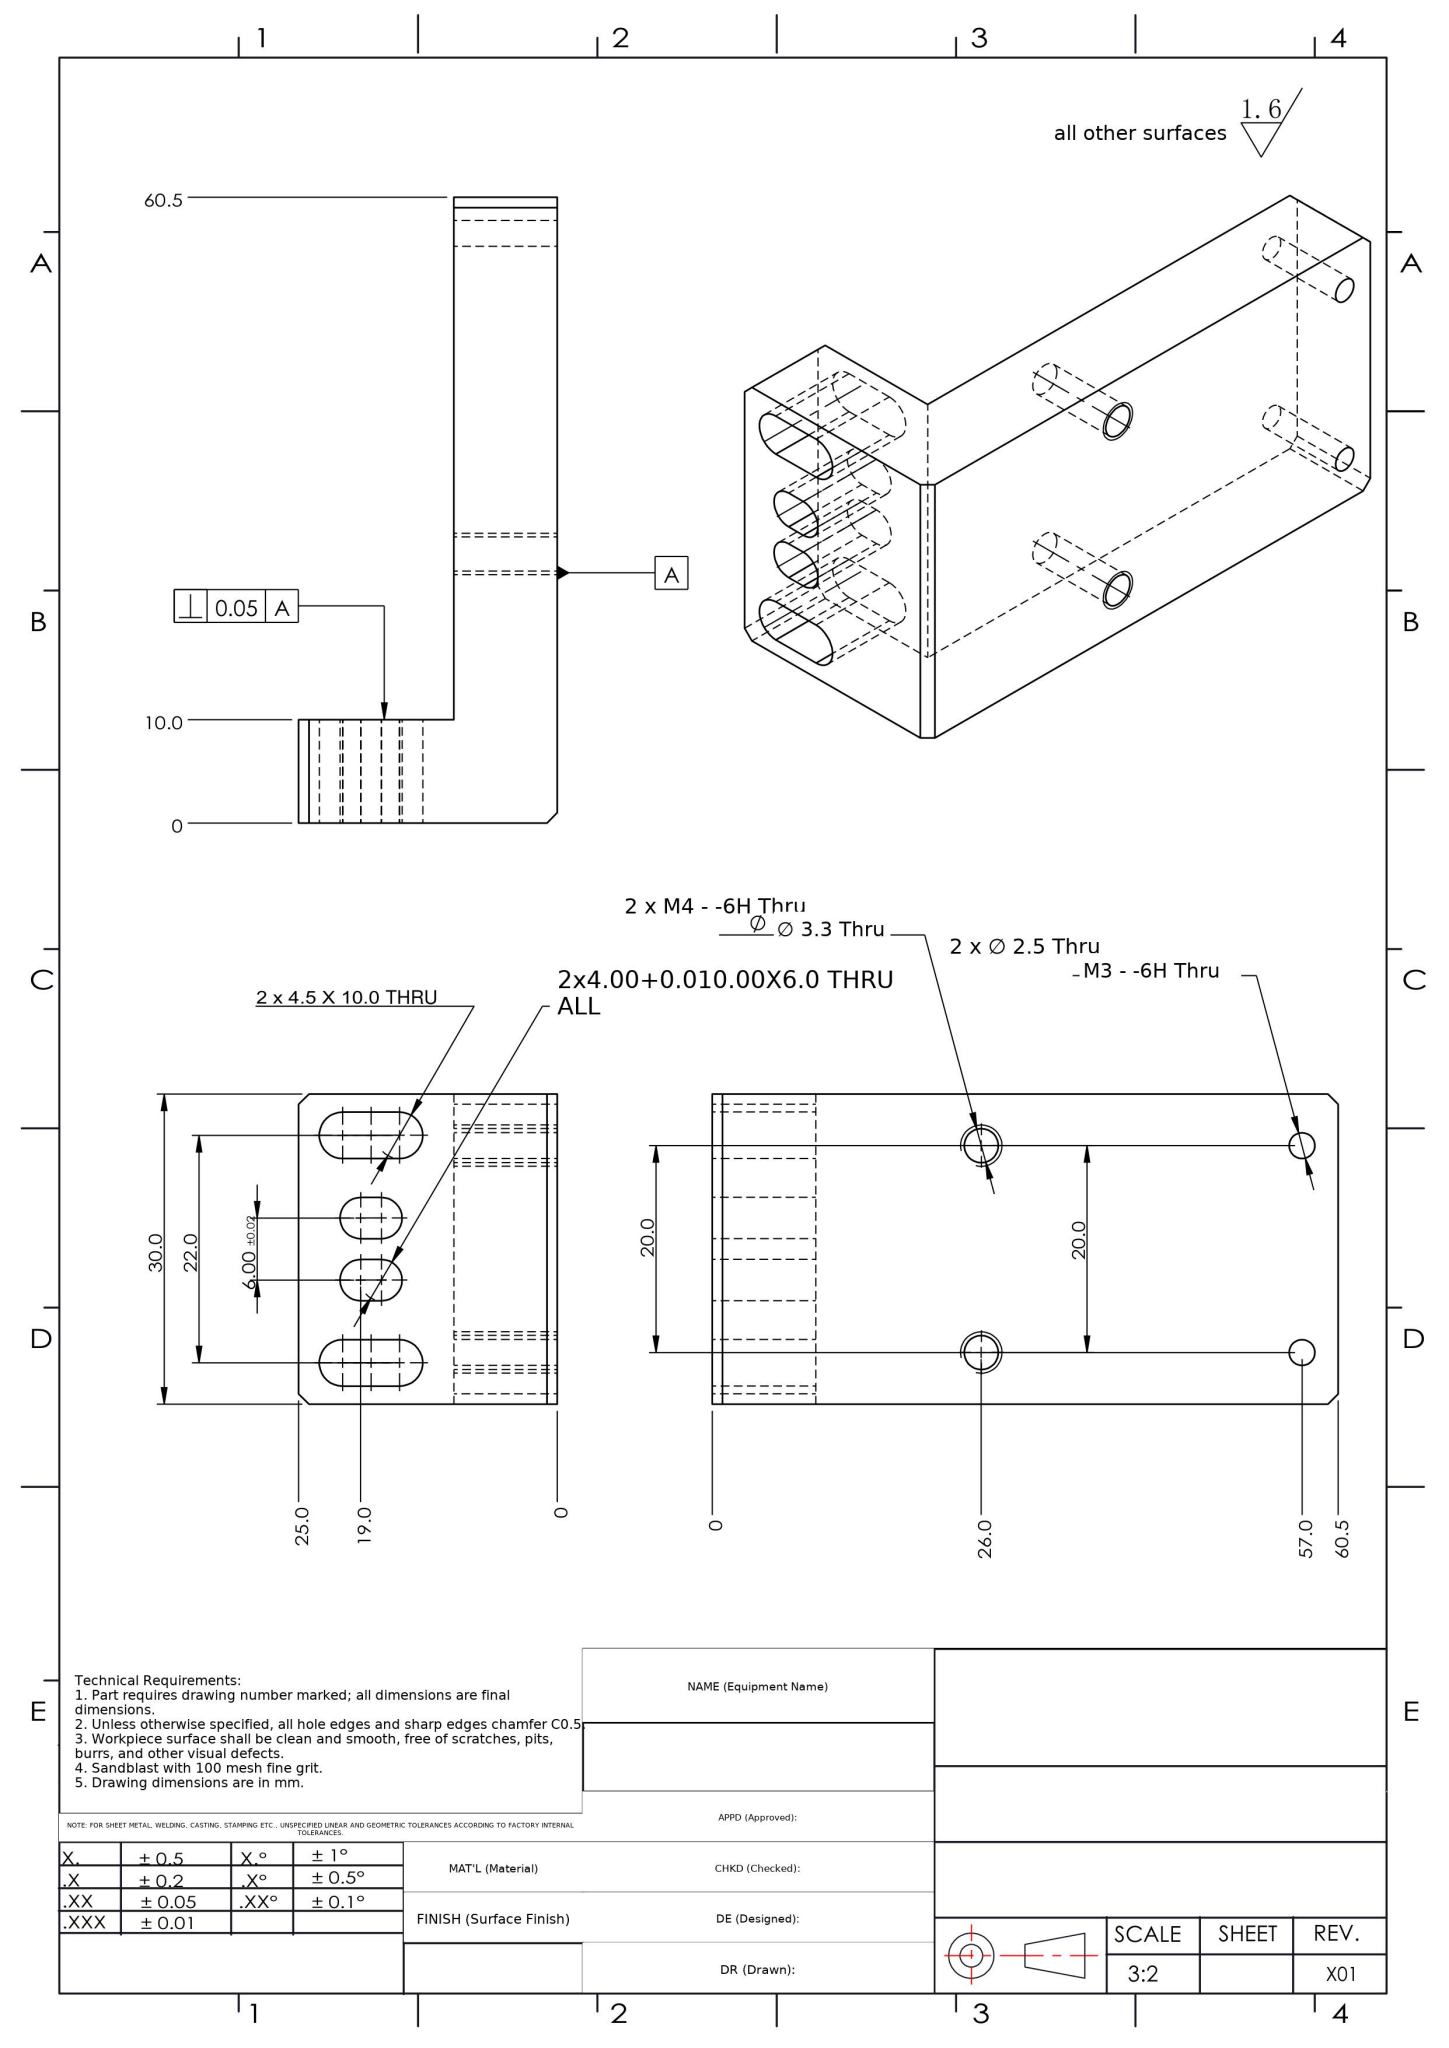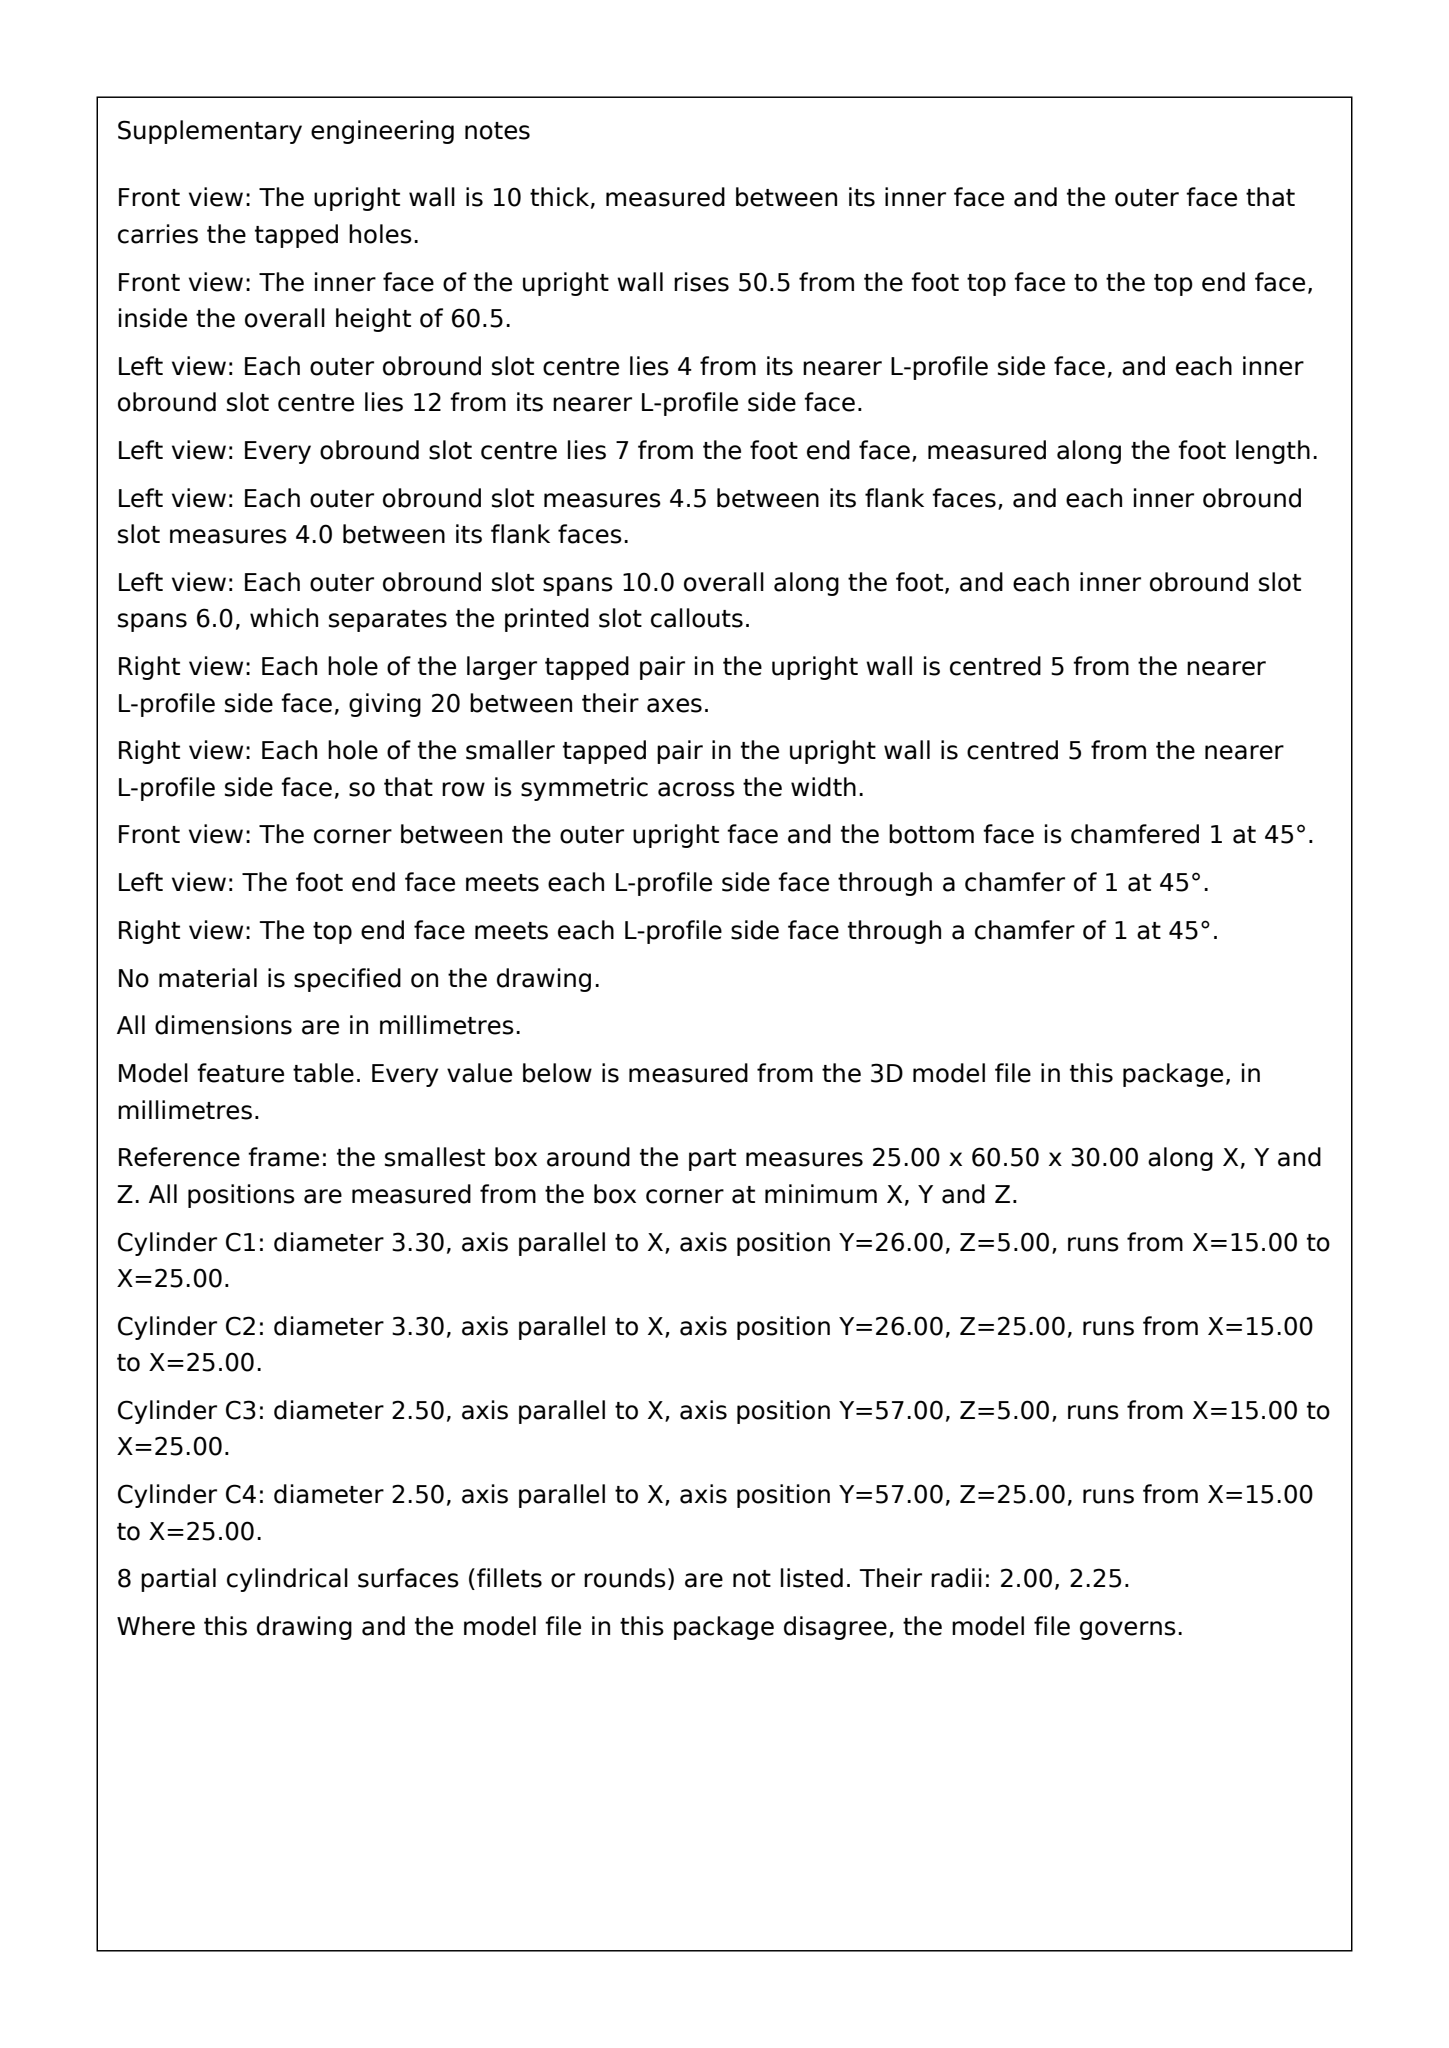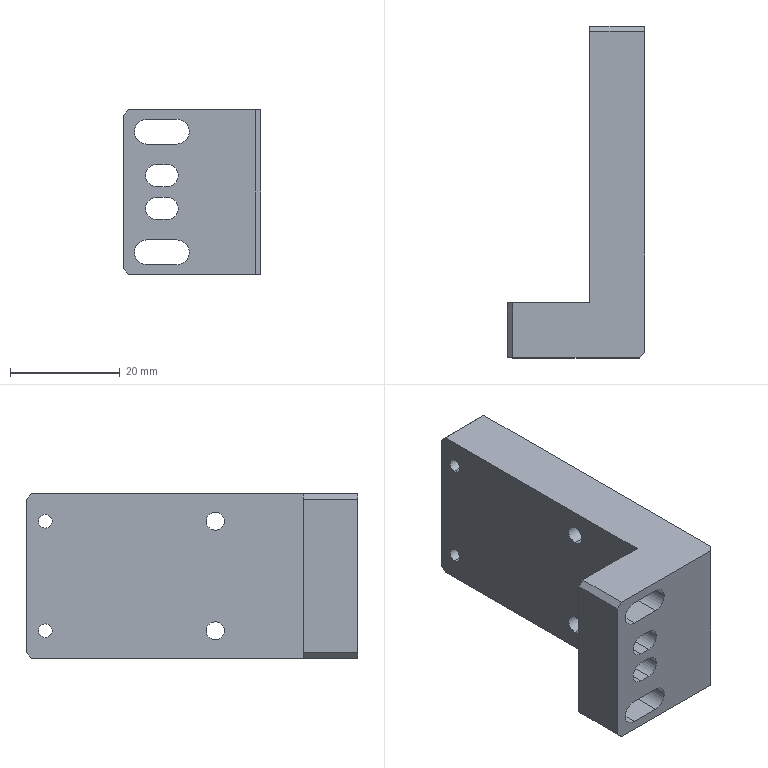Part | SolidWorks | mm | 1 solid | 37 faces | box 25 x 60.5 x 30 mm | volume 21121 mm3 | plane 21 | cylinder 16 | commonest cylinder face diameters 2.5 x4 3.3 x4 4.5 x4 4 x4
Drawing notes:
UPRIGHT LEG 10.0 THK; INNER FACE 15.0 FROM 0 ORD; X-HOLES DP 10.0 | from the solid: Planes x=0/15/25; all Ø3.3 & Ø2.5 cyls axis x, length 10.0 (15.0-25.0)
2 x 4.5 X 10.0 SLOTS: CL 18.0 FROM 0 ORD (ENDS 15.25 & 20.75) | from the solid: Ø4.5 end cyls at x=4.25 & 9.75 => CL x=7.0; 0 ord at x=25 (19.0=Ø4.0 at x=6.0)
M4-6H & Ø2.5/M3-6H ROWS 5.0 FROM EA 30.0 EDGE, SYM ABOUT CL | from the solid: Ø3.3 & Ø2.5 cyls at z=5.0 and z=25.0; part width z=0 to 30.0